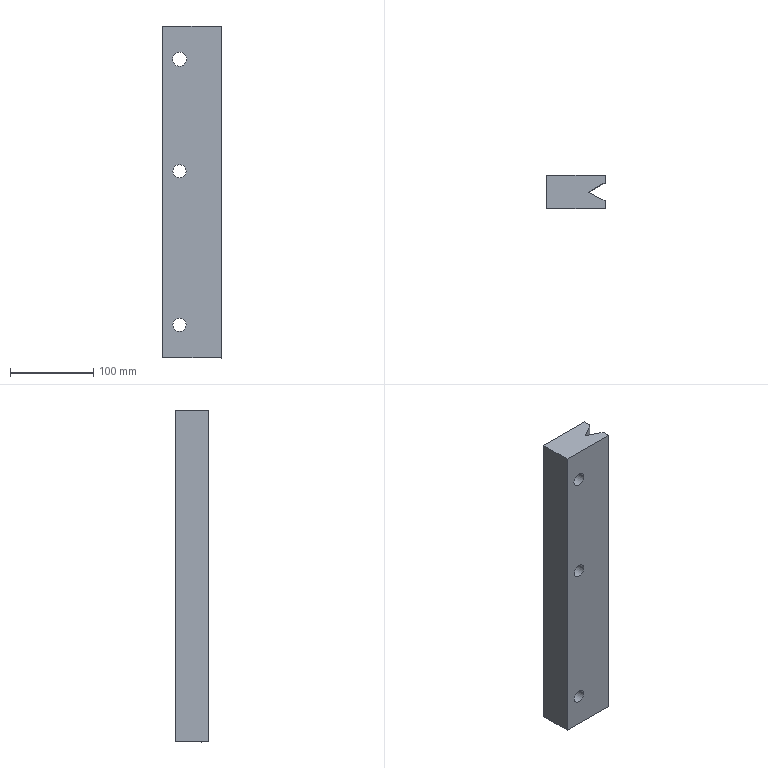Component | SolidWorks | LeftGuideRail-1 | 1 solid | 15 faces | box 70 x 40 x 400 mm | volume 1005616 mm3 | plane 9 | cylinder 6 | commonest cylinder face diameters 16 x4 17 x2
build123d program:
from build123d import *

# Parameters (mm, degrees)
SKETCH1_W                       = 70
SKETCH1_H                       = 400
BOSS_EXTRUDE1_DEPTH             = 40
CUT_EXTRUDE1_DEPTH              = 840.534
DRAFT1_ANGLE                    = 30.559
F_16_0_16_DIAMETER_HOLE1_D      = 16
SKETCH2_R                       = 8.5
REPAIR_SCREWCLEARANCEHOLE_DEPTH = 21


with BuildPart() as part:
    # Sketch1 → Boss-Extrude1 (new body)
    with BuildSketch(Plane(origin=(-632.201, 0, 0), x_dir=(0, 0, -1), z_dir=(1, 0, 0))):
        with Locations((-269.898, 1371.182)):
            Rectangle(SKETCH1_W, SKETCH1_H)
    extrude(amount=-BOSS_EXTRUDE1_DEPTH)

    # Sketch2_2 → Cut-Extrude1 (cut, through all)
    with BuildSketch(Plane(origin=(0, 1571.182, 0), x_dir=(-1, 0, 0), z_dir=(0, 1, 0))):
        Polygon((641.049, 304.898), (641.049, 262.398), (663.354, 304.898), align=None)
    extrude(amount=-CUT_EXTRUDE1_DEPTH, mode=Mode.SUBTRACT)

    # Draft1
    draft1_faces = [part.faces().sort_by_distance(p)[0] for p in [
        (-641.049, 1371.182, 283.648),
    ]]
    draft(draft1_faces, Plane(origin=(-672.201, 1571.182, 304.898), x_dir=(0, 1, 0), z_dir=(0, 0, 1)), DRAFT1_ANGLE)

    # 16.0 _16_ Diameter Hole1 (through all)
    with Locations(Plane.ZY.offset(672.201)):
        with Locations((254.898, 1211.182), (254.898, 1396.182)):
            Hole(F_16_0_16_DIAMETER_HOLE1_D / 2)

    # Sketch2 → Repair_ScrewClearanceHole (cut, symmetric)
    with BuildSketch(Plane(origin=(-652.249, 0, 0), x_dir=(0, 0, -1), z_dir=(1, 0, 0))):
        with Locations((-254.898, 1531.182)):
            Circle(SKETCH2_R)
    extrude(amount=REPAIR_SCREWCLEARANCEHOLE_DEPTH, both=True, mode=Mode.SUBTRACT)


solid = part.part

# Placed as in the assembly
solid = solid.moved(Location((-922.23, 1589.749, -667.519), (90, 90, 0)))
STEP:
#1=COLOUR_RGB('',0.7922,0.8196,0.9333);
#2=FILL_AREA_STYLE_COLOUR('',#1);
#3=FILL_AREA_STYLE('',(#2));
#4=SURFACE_STYLE_FILL_AREA(#3);
#5=SURFACE_SIDE_STYLE('',(#4));
#6=SURFACE_STYLE_USAGE(.BOTH.,#5);
#7=PRESENTATION_STYLE_ASSIGNMENT((#6));
#8=CARTESIAN_POINT('',(-25.938,36.124,34.002));
#9=VERTEX_POINT('',#8);
#10=CARTESIAN_POINT('',(-26.608,36.124,34.002));
#11=VERTEX_POINT('',#10);
#12=CARTESIAN_POINT('',(-26.273,36.124,34.002));
#13=DIRECTION('',(0.,1.,0.));
#14=DIRECTION('',(-1.,0.,0.));
#15=AXIS2_PLACEMENT_3D('',#12,#13,#14);
#16=CIRCLE('',#15,0.3346);
#17=EDGE_CURVE('',#9,#11,#16,.T.);
#18=ORIENTED_EDGE('',*,*,#17,.F.);
#19=CARTESIAN_POINT('',(-25.938,37.699,34.002));
#20=VERTEX_POINT('',#19);
#21=CARTESIAN_POINT('',(-25.938,36.083,34.002));
#22=DIRECTION('',(0.,1.,0.));
#23=VECTOR('',#22,39.37);
#24=LINE('',#21,#23);
#25=EDGE_CURVE('',#9,#20,#24,.T.);
#26=ORIENTED_EDGE('',*,*,#25,.T.);
#27=CARTESIAN_POINT('',(-26.608,37.699,34.002));
#28=VERTEX_POINT('',#27);
#29=CARTESIAN_POINT('',(-26.273,37.699,34.002));
#30=DIRECTION('',(0.,1.,0.));
#31=DIRECTION('',(-1.,0.,0.));
#32=AXIS2_PLACEMENT_3D('',#29,#30,#31);
#33=CIRCLE('',#32,0.3346);
#34=EDGE_CURVE('',#20,#28,#33,.T.);
#35=ORIENTED_EDGE('',*,*,#34,.T.);
#36=CARTESIAN_POINT('',(-26.608,36.083,34.002));
#37=DIRECTION('',(0.,1.,0.));
#38=VECTOR('',#37,39.37);
#39=LINE('',#36,#38);
#40=EDGE_CURVE('',#11,#28,#39,.T.);
#41=ORIENTED_EDGE('',*,*,#40,.F.);
#42=EDGE_LOOP('',(#18,#26,#35,#41));
#43=FACE_OUTER_BOUND('',#42,.T.);
#44=CARTESIAN_POINT('',(-26.273,36.083,34.002));
#45=DIRECTION('',(0.,1.,0.));
#46=DIRECTION('',(-1.,0.,0.));
#47=AXIS2_PLACEMENT_3D('',#44,#45,#46);
#48=CYLINDRICAL_SURFACE('',#47,0.3346);
#49=ADVANCED_FACE('',(#43),#48,.F.);
#50=CARTESIAN_POINT('',(-26.588,37.699,21.404));
#51=VERTEX_POINT('',#50);
#52=CARTESIAN_POINT('',(-25.958,37.699,21.404));
#53=VERTEX_POINT('',#52);
#54=CARTESIAN_POINT('',(-26.273,37.699,21.404));
#55=DIRECTION('',(0.,-1.,0.));
#56=DIRECTION('',(1.,0.,0.));
#57=AXIS2_PLACEMENT_3D('',#54,#55,#56);
#58=CIRCLE('',#57,0.315);
#59=EDGE_CURVE('',#51,#53,#58,.T.);
#60=ORIENTED_EDGE('',*,*,#59,.F.);
#61=CARTESIAN_POINT('',(-26.588,36.124,21.404));
#62=VERTEX_POINT('',#61);
#63=CARTESIAN_POINT('',(-26.588,36.124,21.404));
#64=DIRECTION('',(0.,-1.,0.));
#65=VECTOR('',#64,39.37);
#66=LINE('',#63,#65);
#67=EDGE_CURVE('',#51,#62,#66,.T.);
#68=ORIENTED_EDGE('',*,*,#67,.T.);
#69=CARTESIAN_POINT('',(-25.958,36.124,21.404));
#70=VERTEX_POINT('',#69);
#71=CARTESIAN_POINT('',(-26.273,36.124,21.404));
#72=DIRECTION('',(0.,-1.,0.));
#73=DIRECTION('',(1.,0.,0.));
#74=AXIS2_PLACEMENT_3D('',#71,#72,#73);
#75=CIRCLE('',#74,0.315);
#76=EDGE_CURVE('',#62,#70,#75,.T.);
#77=ORIENTED_EDGE('',*,*,#76,.T.);
#78=CARTESIAN_POINT('',(-25.958,36.124,21.404));
#79=DIRECTION('',(0.,-1.,0.));
#80=VECTOR('',#79,39.37);
#81=LINE('',#78,#80);
#82=EDGE_CURVE('',#53,#70,#81,.T.);
#83=ORIENTED_EDGE('',*,*,#82,.F.);
#84=EDGE_LOOP('',(#60,#68,#77,#83));
#85=FACE_OUTER_BOUND('',#84,.T.);
#86=CARTESIAN_POINT('',(-26.273,36.124,21.404));
#87=DIRECTION('',(0.,-1.,0.));
#88=DIRECTION('',(1.,0.,0.));
#89=AXIS2_PLACEMENT_3D('',#86,#87,#88);
#90=CYLINDRICAL_SURFACE('',#89,0.315);
#91=ADVANCED_FACE('',(#85),#90,.F.);
#92=CARTESIAN_POINT('',(-26.588,37.699,28.688));
#93=VERTEX_POINT('',#92);
#94=CARTESIAN_POINT('',(-25.958,37.699,28.688));
#95=VERTEX_POINT('',#94);
#96=CARTESIAN_POINT('',(-26.273,37.699,28.688));
#97=DIRECTION('',(0.,-1.,0.));
#98=DIRECTION('',(1.,0.,0.));
#99=AXIS2_PLACEMENT_3D('',#96,#97,#98);
#100=CIRCLE('',#99,0.315);
#101=EDGE_CURVE('',#93,#95,#100,.T.);
#102=ORIENTED_EDGE('',*,*,#101,.F.);
#103=CARTESIAN_POINT('',(-26.588,36.124,28.688));
#104=VERTEX_POINT('',#103);
#105=CARTESIAN_POINT('',(-26.588,36.124,28.688));
#106=DIRECTION('',(0.,-1.,0.));
#107=VECTOR('',#106,39.37);
#108=LINE('',#105,#107);
#109=EDGE_CURVE('',#93,#104,#108,.T.);
#110=ORIENTED_EDGE('',*,*,#109,.T.);
#111=CARTESIAN_POINT('',(-25.958,36.124,28.688));
#112=VERTEX_POINT('',#111);
#113=CARTESIAN_POINT('',(-26.273,36.124,28.688));
#114=DIRECTION('',(0.,-1.,0.));
#115=DIRECTION('',(1.,0.,0.));
#116=AXIS2_PLACEMENT_3D('',#113,#114,#115);
#117=CIRCLE('',#116,0.315);
#118=EDGE_CURVE('',#104,#112,#117,.T.);
#119=ORIENTED_EDGE('',*,*,#118,.T.);
#120=CARTESIAN_POINT('',(-25.958,36.124,28.688));
#121=DIRECTION('',(0.,-1.,0.));
#122=VECTOR('',#121,39.37);
#123=LINE('',#120,#122);
#124=EDGE_CURVE('',#95,#112,#123,.T.);
#125=ORIENTED_EDGE('',*,*,#124,.F.);
#126=EDGE_LOOP('',(#102,#110,#119,#125));
#127=FACE_OUTER_BOUND('',#126,.T.);
#128=CARTESIAN_POINT('',(-26.273,36.124,28.688));
#129=DIRECTION('',(0.,-1.,0.));
#130=DIRECTION('',(1.,0.,0.));
#131=AXIS2_PLACEMENT_3D('',#128,#129,#130);
#132=CYLINDRICAL_SURFACE('',#131,0.315);
#133=ADVANCED_FACE('',(#127),#132,.F.);
#134=CARTESIAN_POINT('',(-24.304,36.472,19.829));
#135=VERTEX_POINT('',#134);
#136=CARTESIAN_POINT('',(-24.304,36.472,35.577));
#137=VERTEX_POINT('',#136);
#138=CARTESIAN_POINT('',(-24.304,36.472,19.829));
#139=DIRECTION('',(0.,0.,1.));
#140=VECTOR('',#139,39.37);
#141=LINE('',#138,#140);
#142=EDGE_CURVE('',#135,#137,#141,.T.);
#143=ORIENTED_EDGE('',*,*,#142,.T.);
#144=CARTESIAN_POINT('',(-24.304,36.124,35.577));
#145=VERTEX_POINT('',#144);
#146=CARTESIAN_POINT('',(-24.304,36.124,35.577));
#147=DIRECTION('',(0.,1.,0.));
#148=VECTOR('',#147,39.37);
#149=LINE('',#146,#148);
#150=EDGE_CURVE('',#145,#137,#149,.T.);
#151=ORIENTED_EDGE('',*,*,#150,.F.);
#152=CARTESIAN_POINT('',(-24.304,36.124,19.829));
#153=VERTEX_POINT('',#152);
#154=CARTESIAN_POINT('',(-24.304,36.124,35.577));
#155=DIRECTION('',(-0.,0.,-1.));
#156=VECTOR('',#155,39.37);
#157=LINE('',#154,#156);
#158=EDGE_CURVE('',#145,#153,#157,.T.);
#159=ORIENTED_EDGE('',*,*,#158,.T.);
#160=CARTESIAN_POINT('',(-24.304,36.124,19.829));
#161=DIRECTION('',(0.,1.,0.));
#162=VECTOR('',#161,39.37);
#163=LINE('',#160,#162);
#164=EDGE_CURVE('',#153,#135,#163,.T.);
#165=ORIENTED_EDGE('',*,*,#164,.T.);
#166=EDGE_LOOP('',(#143,#151,#159,#165));
#167=FACE_OUTER_BOUND('',#166,.T.);
#168=CARTESIAN_POINT('',(-24.304,36.124,35.577));
#169=DIRECTION('',(1.,0.,-0.));
#170=DIRECTION('',(-0.,0.,-1.));
#171=AXIS2_PLACEMENT_3D('',#168,#169,#170);
#172=PLANE('',#171);
#173=ADVANCED_FACE('',(#167),#172,.T.);
#174=CARTESIAN_POINT('',(-25.092,36.886,35.577));
#175=VERTEX_POINT('',#174);
#176=CARTESIAN_POINT('',(-25.978,37.35,35.577));
#177=DIRECTION('',(0.8855,-0.4647,-0.));
#178=VECTOR('',#177,39.37);
#179=LINE('',#176,#178);
#180=EDGE_CURVE('',#175,#137,#179,.T.);
#181=ORIENTED_EDGE('',*,*,#180,.F.);
#182=CARTESIAN_POINT('',(-24.304,37.35,35.577));
#183=VERTEX_POINT('',#182);
#184=CARTESIAN_POINT('',(-26.885,35.827,35.577));
#185=DIRECTION('',(-0.8611,-0.5084,0.));
#186=VECTOR('',#185,39.37);
#187=LINE('',#184,#186);
#188=EDGE_CURVE('',#183,#175,#187,.T.);
#189=ORIENTED_EDGE('',*,*,#188,.F.);
#190=CARTESIAN_POINT('',(-24.304,37.699,35.577));
#191=VERTEX_POINT('',#190);
#192=CARTESIAN_POINT('',(-24.304,36.124,35.577));
#193=DIRECTION('',(0.,1.,0.));
#194=VECTOR('',#193,39.37);
#195=LINE('',#192,#194);
#196=EDGE_CURVE('',#183,#191,#195,.T.);
#197=ORIENTED_EDGE('',*,*,#196,.T.);
#198=CARTESIAN_POINT('',(-27.06,37.699,35.577));
#199=VERTEX_POINT('',#198);
#200=CARTESIAN_POINT('',(-27.06,37.699,35.577));
#201=DIRECTION('',(1.,0.,-0.));
#202=VECTOR('',#201,39.37);
#203=LINE('',#200,#202);
#204=EDGE_CURVE('',#199,#191,#203,.T.);
#205=ORIENTED_EDGE('',*,*,#204,.F.);
#206=CARTESIAN_POINT('',(-27.06,36.124,35.577));
#207=VERTEX_POINT('',#206);
#208=CARTESIAN_POINT('',(-27.06,36.124,35.577));
#209=DIRECTION('',(0.,1.,0.));
#210=VECTOR('',#209,39.37);
#211=LINE('',#208,#210);
#212=EDGE_CURVE('',#207,#199,#211,.T.);
#213=ORIENTED_EDGE('',*,*,#212,.F.);
#214=CARTESIAN_POINT('',(-27.06,36.124,35.577));
#215=DIRECTION('',(1.,0.,-0.));
#216=VECTOR('',#215,39.37);
#217=LINE('',#214,#216);
#218=EDGE_CURVE('',#207,#145,#217,.T.);
#219=ORIENTED_EDGE('',*,*,#218,.T.);
#220=ORIENTED_EDGE('',*,*,#150,.T.);
#221=EDGE_LOOP('',(#181,#189,#197,#205,#213,#219,#220));
#222=FACE_OUTER_BOUND('',#221,.T.);
#223=CARTESIAN_POINT('',(-27.06,36.124,35.577));
#224=DIRECTION('',(0.,0.,1.));
#225=DIRECTION('',(1.,0.,-0.));
#226=AXIS2_PLACEMENT_3D('',#223,#224,#225);
#227=PLANE('',#226);
#228=ADVANCED_FACE('',(#222),#227,.T.);
#229=CARTESIAN_POINT('',(-27.06,37.699,19.829));
#230=VERTEX_POINT('',#229);
#231=CARTESIAN_POINT('',(-27.06,37.699,19.829));
#232=DIRECTION('',(0.,0.,1.));
#233=VECTOR('',#232,39.37);
#234=LINE('',#231,#233);
#235=EDGE_CURVE('',#230,#199,#234,.T.);
#236=ORIENTED_EDGE('',*,*,#235,.F.);
#237=CARTESIAN_POINT('',(-27.06,36.124,19.829));
#238=VERTEX_POINT('',#237);
#239=CARTESIAN_POINT('',(-27.06,36.124,19.829));
#240=DIRECTION('',(0.,1.,0.));
#241=VECTOR('',#240,39.37);
#242=LINE('',#239,#241);
#243=EDGE_CURVE('',#238,#230,#242,.T.);
#244=ORIENTED_EDGE('',*,*,#243,.F.);
#245=CARTESIAN_POINT('',(-27.06,36.124,19.829));
#246=DIRECTION('',(0.,0.,1.));
#247=VECTOR('',#246,39.37);
#248=LINE('',#245,#247);
#249=EDGE_CURVE('',#238,#207,#248,.T.);
#250=ORIENTED_EDGE('',*,*,#249,.T.);
#251=ORIENTED_EDGE('',*,*,#212,.T.);
#252=EDGE_LOOP('',(#236,#244,#250,#251));
#253=FACE_OUTER_BOUND('',#252,.T.);
#254=CARTESIAN_POINT('',(-27.06,36.124,19.829));
#255=DIRECTION('',(-1.,0.,0.));
#256=DIRECTION('',(0.,-1.,0.));
#257=AXIS2_PLACEMENT_3D('',#254,#255,#256);
#258=PLANE('',#257);
#259=ADVANCED_FACE('',(#253),#258,.T.);
#260=CARTESIAN_POINT('',(-25.092,36.886,19.829));
#261=VERTEX_POINT('',#260);
#262=CARTESIAN_POINT('',(-25.978,37.35,19.829));
#263=DIRECTION('',(0.8855,-0.4647,-0.));
#264=VECTOR('',#263,39.37);
#265=LINE('',#262,#264);
#266=EDGE_CURVE('',#261,#135,#265,.T.);
#267=ORIENTED_EDGE('',*,*,#266,.T.);
#268=ORIENTED_EDGE('',*,*,#164,.F.);
#269=CARTESIAN_POINT('',(-24.304,36.124,19.829));
#270=DIRECTION('',(-1.,0.,0.));
#271=VECTOR('',#270,39.37);
#272=LINE('',#269,#271);
#273=EDGE_CURVE('',#153,#238,#272,.T.);
#274=ORIENTED_EDGE('',*,*,#273,.T.);
#275=ORIENTED_EDGE('',*,*,#243,.T.);
#276=CARTESIAN_POINT('',(-24.304,37.699,19.829));
#277=VERTEX_POINT('',#276);
#278=CARTESIAN_POINT('',(-24.304,37.699,19.829));
#279=DIRECTION('',(-1.,0.,0.));
#280=VECTOR('',#279,39.37);
#281=LINE('',#278,#280);
#282=EDGE_CURVE('',#277,#230,#281,.T.);
#283=ORIENTED_EDGE('',*,*,#282,.F.);
#284=CARTESIAN_POINT('',(-24.304,37.35,19.829));
#285=VERTEX_POINT('',#284);
#286=CARTESIAN_POINT('',(-24.304,36.124,19.829));
#287=DIRECTION('',(0.,1.,0.));
#288=VECTOR('',#287,39.37);
#289=LINE('',#286,#288);
#290=EDGE_CURVE('',#285,#277,#289,.T.);
#291=ORIENTED_EDGE('',*,*,#290,.F.);
#292=CARTESIAN_POINT('',(-24.304,37.35,19.829));
#293=DIRECTION('',(-0.8611,-0.5084,0.));
#294=VECTOR('',#293,39.37);
#295=LINE('',#292,#294);
#296=EDGE_CURVE('',#285,#261,#295,.T.);
#297=ORIENTED_EDGE('',*,*,#296,.T.);
#298=EDGE_LOOP('',(#267,#268,#274,#275,#283,#291,#297));
#299=FACE_OUTER_BOUND('',#298,.T.);
#300=CARTESIAN_POINT('',(-24.304,36.124,19.829));
#301=DIRECTION('',(0.,0.,-1.));
#302=DIRECTION('',(-1.,0.,0.));
#303=AXIS2_PLACEMENT_3D('',#300,#301,#302);
#304=PLANE('',#303);
#305=ADVANCED_FACE('',(#299),#304,.T.);
#306=CARTESIAN_POINT('',(-24.304,37.35,19.829));
#307=DIRECTION('',(0.,0.,1.));
#308=VECTOR('',#307,39.37);
#309=LINE('',#306,#308);
#310=EDGE_CURVE('',#285,#183,#309,.T.);
#311=ORIENTED_EDGE('',*,*,#310,.F.);
#312=ORIENTED_EDGE('',*,*,#290,.T.);
#313=CARTESIAN_POINT('',(-24.304,37.699,35.577));
#314=DIRECTION('',(-0.,0.,-1.));
#315=VECTOR('',#314,39.37);
#316=LINE('',#313,#315);
#317=EDGE_CURVE('',#191,#277,#316,.T.);
#318=ORIENTED_EDGE('',*,*,#317,.F.);
#319=ORIENTED_EDGE('',*,*,#196,.F.);
#320=EDGE_LOOP('',(#311,#312,#318,#319));
#321=FACE_OUTER_BOUND('',#320,.T.);
#322=CARTESIAN_POINT('',(-24.304,36.124,35.577));
#323=DIRECTION('',(1.,0.,-0.));
#324=DIRECTION('',(-0.,0.,-1.));
#325=AXIS2_PLACEMENT_3D('',#322,#323,#324);
#326=PLANE('',#325);
#327=ADVANCED_FACE('',(#321),#326,.T.);
#328=CARTESIAN_POINT('',(-26.273,36.124,34.002));
#329=DIRECTION('',(0.,1.,0.));
#330=DIRECTION('',(-1.,0.,0.));
#331=AXIS2_PLACEMENT_3D('',#328,#329,#330);
#332=CIRCLE('',#331,0.3346);
#333=EDGE_CURVE('',#11,#9,#332,.T.);
#334=ORIENTED_EDGE('',*,*,#333,.T.);
#335=ORIENTED_EDGE('',*,*,#17,.T.);
#336=EDGE_LOOP('',(#334,#335));
#337=FACE_BOUND('',#336,.T.);
#338=CARTESIAN_POINT('',(-26.273,36.124,21.404));
#339=DIRECTION('',(0.,-1.,0.));
#340=DIRECTION('',(1.,0.,0.));
#341=AXIS2_PLACEMENT_3D('',#338,#339,#340);
#342=CIRCLE('',#341,0.315);
#343=EDGE_CURVE('',#70,#62,#342,.T.);
#344=ORIENTED_EDGE('',*,*,#343,.F.);
#345=ORIENTED_EDGE('',*,*,#76,.F.);
#346=EDGE_LOOP('',(#344,#345));
#347=FACE_BOUND('',#346,.T.);
#348=CARTESIAN_POINT('',(-26.273,36.124,28.688));
#349=DIRECTION('',(0.,-1.,0.));
#350=DIRECTION('',(1.,0.,0.));
#351=AXIS2_PLACEMENT_3D('',#348,#349,#350);
#352=CIRCLE('',#351,0.315);
#353=EDGE_CURVE('',#112,#104,#352,.T.);
#354=ORIENTED_EDGE('',*,*,#353,.F.);
#355=ORIENTED_EDGE('',*,*,#118,.F.);
#356=EDGE_LOOP('',(#354,#355));
#357=FACE_BOUND('',#356,.T.);
#358=ORIENTED_EDGE('',*,*,#218,.F.);
#359=ORIENTED_EDGE('',*,*,#249,.F.);
#360=ORIENTED_EDGE('',*,*,#273,.F.);
#361=ORIENTED_EDGE('',*,*,#158,.F.);
#362=EDGE_LOOP('',(#358,#359,#360,#361));
#363=FACE_OUTER_BOUND('',#362,.T.);
#364=CARTESIAN_POINT('',(-36.308,36.124,-26.28));
#365=DIRECTION('',(0.,1.,0.));
#366=DIRECTION('',(-1.,0.,0.));
#367=AXIS2_PLACEMENT_3D('',#364,#365,#366);
#368=PLANE('',#367);
#369=ADVANCED_FACE('',(#337,#347,#357,#363),#368,.F.);
#370=CARTESIAN_POINT('',(-26.273,37.699,34.002));
#371=DIRECTION('',(0.,1.,0.));
#372=DIRECTION('',(-1.,0.,0.));
#373=AXIS2_PLACEMENT_3D('',#370,#371,#372);
#374=CIRCLE('',#373,0.3346);
#375=EDGE_CURVE('',#28,#20,#374,.T.);
#376=ORIENTED_EDGE('',*,*,#375,.F.);
#377=ORIENTED_EDGE('',*,*,#34,.F.);
#378=EDGE_LOOP('',(#376,#377));
#379=FACE_BOUND('',#378,.T.);
#380=CARTESIAN_POINT('',(-26.273,37.699,21.404));
#381=DIRECTION('',(0.,-1.,0.));
#382=DIRECTION('',(1.,0.,0.));
#383=AXIS2_PLACEMENT_3D('',#380,#381,#382);
#384=CIRCLE('',#383,0.315);
#385=EDGE_CURVE('',#53,#51,#384,.T.);
#386=ORIENTED_EDGE('',*,*,#385,.T.);
#387=ORIENTED_EDGE('',*,*,#59,.T.);
#388=EDGE_LOOP('',(#386,#387));
#389=FACE_BOUND('',#388,.T.);
#390=CARTESIAN_POINT('',(-26.273,37.699,28.688));
#391=DIRECTION('',(0.,-1.,0.));
#392=DIRECTION('',(1.,0.,0.));
#393=AXIS2_PLACEMENT_3D('',#390,#391,#392);
#394=CIRCLE('',#393,0.315);
#395=EDGE_CURVE('',#95,#93,#394,.T.);
#396=ORIENTED_EDGE('',*,*,#395,.T.);
#397=ORIENTED_EDGE('',*,*,#101,.T.);
#398=EDGE_LOOP('',(#396,#397));
#399=FACE_BOUND('',#398,.T.);
#400=ORIENTED_EDGE('',*,*,#204,.T.);
#401=ORIENTED_EDGE('',*,*,#317,.T.);
#402=ORIENTED_EDGE('',*,*,#282,.T.);
#403=ORIENTED_EDGE('',*,*,#235,.T.);
#404=EDGE_LOOP('',(#400,#401,#402,#403));
#405=FACE_OUTER_BOUND('',#404,.T.);
#406=CARTESIAN_POINT('',(-36.308,37.699,-26.28));
#407=DIRECTION('',(0.,1.,0.));
#408=DIRECTION('',(-1.,0.,0.));
#409=AXIS2_PLACEMENT_3D('',#406,#407,#408);
#410=PLANE('',#409);
#411=ADVANCED_FACE('',(#379,#389,#399,#405),#410,.T.);
#412=ORIENTED_EDGE('',*,*,#180,.T.);
#413=ORIENTED_EDGE('',*,*,#142,.F.);
#414=ORIENTED_EDGE('',*,*,#266,.F.);
#415=CARTESIAN_POINT('',(-25.092,36.886,19.829));
#416=DIRECTION('',(0.,-0.,1.));
#417=VECTOR('',#416,39.37);
#418=LINE('',#415,#417);
#419=EDGE_CURVE('',#261,#175,#418,.T.);
#420=ORIENTED_EDGE('',*,*,#419,.T.);
#421=EDGE_LOOP('',(#412,#413,#414,#420));
#422=FACE_OUTER_BOUND('',#421,.T.);
#423=CARTESIAN_POINT('',(-25.978,37.35,19.829));
#424=DIRECTION('',(-0.4647,-0.8855,0.));
#425=DIRECTION('',(0.8855,-0.4647,0.));
#426=AXIS2_PLACEMENT_3D('',#423,#424,#425);
#427=PLANE('',#426);
#428=ADVANCED_FACE('',(#422),#427,.F.);
#429=ORIENTED_EDGE('',*,*,#188,.T.);
#430=ORIENTED_EDGE('',*,*,#419,.F.);
#431=ORIENTED_EDGE('',*,*,#296,.F.);
#432=ORIENTED_EDGE('',*,*,#310,.T.);
#433=EDGE_LOOP('',(#429,#430,#431,#432));
#434=FACE_OUTER_BOUND('',#433,.T.);
#435=CARTESIAN_POINT('',(-24.304,37.35,19.829));
#436=DIRECTION('',(0.5084,-0.8611,-0.));
#437=DIRECTION('',(0.8611,0.5084,0.));
#438=AXIS2_PLACEMENT_3D('',#435,#436,#437);
#439=PLANE('',#438);
#440=ADVANCED_FACE('',(#434),#439,.T.);
#441=ORIENTED_EDGE('',*,*,#109,.F.);
#442=ORIENTED_EDGE('',*,*,#395,.F.);
#443=ORIENTED_EDGE('',*,*,#124,.T.);
#444=ORIENTED_EDGE('',*,*,#353,.T.);
#445=EDGE_LOOP('',(#441,#442,#443,#444));
#446=FACE_OUTER_BOUND('',#445,.T.);
#447=CARTESIAN_POINT('',(-26.273,36.124,28.688));
#448=DIRECTION('',(0.,-1.,0.));
#449=DIRECTION('',(1.,0.,0.));
#450=AXIS2_PLACEMENT_3D('',#447,#448,#449);
#451=CYLINDRICAL_SURFACE('',#450,0.315);
#452=ADVANCED_FACE('',(#446),#451,.F.);
#453=ORIENTED_EDGE('',*,*,#67,.F.);
#454=ORIENTED_EDGE('',*,*,#385,.F.);
#455=ORIENTED_EDGE('',*,*,#82,.T.);
#456=ORIENTED_EDGE('',*,*,#343,.T.);
#457=EDGE_LOOP('',(#453,#454,#455,#456));
#458=FACE_OUTER_BOUND('',#457,.T.);
#459=CARTESIAN_POINT('',(-26.273,36.124,21.404));
#460=DIRECTION('',(0.,-1.,0.));
#461=DIRECTION('',(1.,0.,0.));
#462=AXIS2_PLACEMENT_3D('',#459,#460,#461);
#463=CYLINDRICAL_SURFACE('',#462,0.315);
#464=ADVANCED_FACE('',(#458),#463,.F.);
#465=ORIENTED_EDGE('',*,*,#25,.F.);
#466=ORIENTED_EDGE('',*,*,#333,.F.);
#467=ORIENTED_EDGE('',*,*,#40,.T.);
#468=ORIENTED_EDGE('',*,*,#375,.T.);
#469=EDGE_LOOP('',(#465,#466,#467,#468));
#470=FACE_OUTER_BOUND('',#469,.T.);
#471=CARTESIAN_POINT('',(-26.273,36.083,34.002));
#472=DIRECTION('',(0.,1.,0.));
#473=DIRECTION('',(-1.,0.,0.));
#474=AXIS2_PLACEMENT_3D('',#471,#472,#473);
#475=CYLINDRICAL_SURFACE('',#474,0.3346);
#476=ADVANCED_FACE('',(#470),#475,.F.);
#477=CLOSED_SHELL('',(#49,#91,#133,#173,#228,#259,#305,#327,#369,#411,#428,#440,#452,#464,#476));
#478=MANIFOLD_SOLID_BREP('',#477);
#479=STYLED_ITEM('',(#7),#478);
#480=(LENGTH_UNIT()NAMED_UNIT(*)SI_UNIT($,.METRE.));
#481=LENGTH_MEASURE_WITH_UNIT(LENGTH_MEASURE(0.0254),#480);
#482=DIMENSIONAL_EXPONENTS(1.,0.,0.,0.,0.,0.,0.);
#483=(CONVERSION_BASED_UNIT('',#481)LENGTH_UNIT()NAMED_UNIT(#482));
#484=UNCERTAINTY_MEASURE_WITH_UNIT(LENGTH_MEASURE(0.00001),#483,'','');
#485=(NAMED_UNIT(*)PLANE_ANGLE_UNIT()SI_UNIT($,.RADIAN.));
#486=(NAMED_UNIT(*)SI_UNIT($,.STERADIAN.)SOLID_ANGLE_UNIT());
#487=(GEOMETRIC_REPRESENTATION_CONTEXT(3)GLOBAL_UNCERTAINTY_ASSIGNED_CONTEXT((#484))GLOBAL_UNIT_ASSIGNED_CONTEXT((#483,#485,#486))REPRESENTATION_CONTEXT('',''));
#488=MECHANICAL_DESIGN_GEOMETRIC_PRESENTATION_REPRESENTATION('',(#479),#487);
#489=CARTESIAN_POINT('',(0.,0.,0.));
#490=DIRECTION('',(0.,0.,1.));
#491=DIRECTION('',(1.,0.,0.));
#492=AXIS2_PLACEMENT_3D('',#489,#490,#491);
#493=(LENGTH_UNIT()NAMED_UNIT(*)SI_UNIT($,.METRE.));
#494=LENGTH_MEASURE_WITH_UNIT(LENGTH_MEASURE(0.0254),#493);
#495=DIMENSIONAL_EXPONENTS(1.,0.,0.,0.,0.,0.,0.);
#496=(CONVERSION_BASED_UNIT('',#494)LENGTH_UNIT()NAMED_UNIT(#495));
#497=UNCERTAINTY_MEASURE_WITH_UNIT(LENGTH_MEASURE(0.00001),#496,'','');
#498=(NAMED_UNIT(*)PLANE_ANGLE_UNIT()SI_UNIT($,.RADIAN.));
#499=(NAMED_UNIT(*)SI_UNIT($,.STERADIAN.)SOLID_ANGLE_UNIT());
#500=(GEOMETRIC_REPRESENTATION_CONTEXT(3)GLOBAL_UNCERTAINTY_ASSIGNED_CONTEXT((#497))GLOBAL_UNIT_ASSIGNED_CONTEXT((#496,#498,#499))REPRESENTATION_CONTEXT('',''));
#501=ADVANCED_BREP_SHAPE_REPRESENTATION('',(#478,#492),#500);
#502=PRESENTATION_LAYER_ASSIGNMENT('','',(#479));